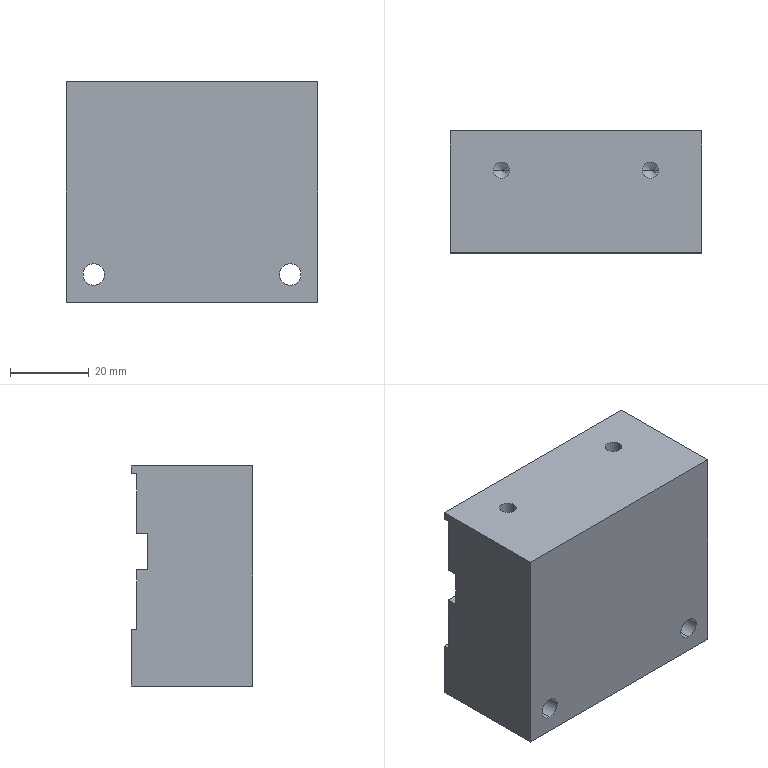Component | SolidWorks | JCT-03-01Base-1 | 1 solid | 32 faces | box 64 x 31 x 56 mm | volume 103150 mm3 | plane 16 | cylinder 12 | cone 4 | commonest cylinder face diameters 4.2 x4 10 x4 5.5 x4
build123d program:
from build123d import *

# Parameters (mm, degrees)
EXTRUDE1_DEPTH                                  = 32
M5_HEX_SOCKET_HEAD_CAP_SCREW_CBORE1_D           = 5.5
M5_HEX_SOCKET_HEAD_CAP_SCREW_CBORE1_CBORE_D     = 10
M5_HEX_SOCKET_HEAD_CAP_SCREW_CBORE1_CBORE_DEPTH = 6
M5_TAPPED_HOLE1_D                               = 4.2
M5_TAPPED_HOLE1_DEPTH                           = 12.4
M5_TAPPED_HOLE1_TIP                             = 1.262


with BuildPart() as part:
    # Sketch1 → Extrude1 (new, symmetric)
    with BuildSketch(Plane(origin=(0, 0, 0), x_dir=(0, 0, -1), z_dir=(1, 0, 0))):
        Polygon((0, 0), (-56, 0), (-56, 31), (-54, 31), (-54, 29.5), (-38.85, 29.5), (-38.85, 26.7), (-29.55, 26.7), (-29.55, 29.5), (-14.4, 29.5), (-14.4, 31), (0, 31), align=None)
    extrude(amount=EXTRUDE1_DEPTH, both=True)

    # M5 Hex Socket Head Cap Screw CBORE1 (through all)
    with Locations(Plane(origin=(0, 31, 0), x_dir=(-1, 0, 0), z_dir=(0, 1, 0))):
        with Locations((25, 7), (-25, 7)):
            CounterBoreHole(M5_HEX_SOCKET_HEAD_CAP_SCREW_CBORE1_D / 2, M5_HEX_SOCKET_HEAD_CAP_SCREW_CBORE1_CBORE_D / 2, M5_HEX_SOCKET_HEAD_CAP_SCREW_CBORE1_CBORE_DEPTH)

    # M5 Tapped Hole1
    with Locations(Plane.XY.offset(56)):
        with Locations((-19, 21), (19, 21)):
            Hole(M5_TAPPED_HOLE1_D / 2, depth=M5_TAPPED_HOLE1_DEPTH)
            with Locations((0, 0, -(M5_TAPPED_HOLE1_DEPTH + M5_TAPPED_HOLE1_TIP / 2))):  # 118° drill point
                Cone(0, M5_TAPPED_HOLE1_D / 2, M5_TAPPED_HOLE1_TIP, mode=Mode.SUBTRACT)


solid = part.part

# Placed as in the assembly
solid = solid.moved(Location((4.266, -17.701, 0), (0, 0, 0)))
STEP:
#1=COLOUR_RGB('',0.7922,0.8196,0.9333);
#2=FILL_AREA_STYLE_COLOUR('',#1);
#3=FILL_AREA_STYLE('',(#2));
#4=SURFACE_STYLE_FILL_AREA(#3);
#5=SURFACE_SIDE_STYLE('',(#4));
#6=SURFACE_STYLE_USAGE(.BOTH.,#5);
#7=PRESENTATION_STYLE_ASSIGNMENT((#6));
#8=CARTESIAN_POINT('',(-0.6627,0.1299,1.717));
#9=VERTEX_POINT('',#8);
#10=CARTESIAN_POINT('',(-0.4974,0.1299,1.717));
#11=VERTEX_POINT('',#10);
#12=CARTESIAN_POINT('',(-0.5801,0.1299,1.717));
#13=DIRECTION('',(0.,0.,1.));
#14=DIRECTION('',(1.,0.,0.));
#15=AXIS2_PLACEMENT_3D('',#12,#13,#14);
#16=CIRCLE('',#15,0.08268);
#17=EDGE_CURVE('',#9,#11,#16,.T.);
#18=ORIENTED_EDGE('',*,*,#17,.F.);
#19=CARTESIAN_POINT('',(-0.6627,0.1299,2.205));
#20=VERTEX_POINT('',#19);
#21=CARTESIAN_POINT('',(-0.6627,0.1299,2.205));
#22=DIRECTION('',(0.,0.,1.));
#23=VECTOR('',#22,39.37);
#24=LINE('',#21,#23);
#25=EDGE_CURVE('',#9,#20,#24,.T.);
#26=ORIENTED_EDGE('',*,*,#25,.T.);
#27=CARTESIAN_POINT('',(-0.4974,0.1299,2.205));
#28=VERTEX_POINT('',#27);
#29=CARTESIAN_POINT('',(-0.5801,0.1299,2.205));
#30=DIRECTION('',(0.,0.,1.));
#31=DIRECTION('',(1.,0.,0.));
#32=AXIS2_PLACEMENT_3D('',#29,#30,#31);
#33=CIRCLE('',#32,0.08268);
#34=EDGE_CURVE('',#20,#28,#33,.T.);
#35=ORIENTED_EDGE('',*,*,#34,.T.);
#36=CARTESIAN_POINT('',(-0.4974,0.1299,2.205));
#37=DIRECTION('',(0.,0.,1.));
#38=VECTOR('',#37,39.37);
#39=LINE('',#36,#38);
#40=EDGE_CURVE('',#11,#28,#39,.T.);
#41=ORIENTED_EDGE('',*,*,#40,.F.);
#42=EDGE_LOOP('',(#18,#26,#35,#41));
#43=FACE_OUTER_BOUND('',#42,.T.);
#44=CARTESIAN_POINT('',(-0.5801,0.1299,2.205));
#45=DIRECTION('',(0.,0.,1.));
#46=DIRECTION('',(1.,0.,0.));
#47=AXIS2_PLACEMENT_3D('',#44,#45,#46);
#48=CYLINDRICAL_SURFACE('',#47,0.08268);
#49=ADVANCED_FACE('',(#43),#48,.F.);
#50=CARTESIAN_POINT('',(-0.5801,0.1299,1.667));
#51=VERTEX_POINT('',#50);
#52=CARTESIAN_POINT('',(-0.4974,0.1299,1.717));
#53=DIRECTION('',(0.8572,0.,0.515));
#54=VECTOR('',#53,39.37);
#55=LINE('',#52,#54);
#56=EDGE_CURVE('',#51,#11,#55,.T.);
#57=ORIENTED_EDGE('',*,*,#56,.F.);
#58=CARTESIAN_POINT('',(-0.6627,0.1299,1.717));
#59=DIRECTION('',(-0.8572,0.,0.515));
#60=VECTOR('',#59,39.37);
#61=LINE('',#58,#60);
#62=EDGE_CURVE('',#51,#9,#61,.T.);
#63=ORIENTED_EDGE('',*,*,#62,.T.);
#64=ORIENTED_EDGE('',*,*,#17,.T.);
#65=EDGE_LOOP('',(#57,#63,#64));
#66=FACE_OUTER_BOUND('',#65,.T.);
#67=CARTESIAN_POINT('',(-0.5801,0.1299,1.717));
#68=DIRECTION('',(0.,0.,1.));
#69=DIRECTION('',(1.,0.,0.));
#70=AXIS2_PLACEMENT_3D('',#67,#68,#69);
#71=CONICAL_SURFACE('',#70,0.08268,1.03);
#72=ADVANCED_FACE('',(#66),#71,.F.);
#73=CARTESIAN_POINT('',(0.8333,0.1299,1.717));
#74=VERTEX_POINT('',#73);
#75=CARTESIAN_POINT('',(0.9987,0.1299,1.717));
#76=VERTEX_POINT('',#75);
#77=CARTESIAN_POINT('',(0.916,0.1299,1.717));
#78=DIRECTION('',(0.,0.,1.));
#79=DIRECTION('',(1.,0.,0.));
#80=AXIS2_PLACEMENT_3D('',#77,#78,#79);
#81=CIRCLE('',#80,0.08268);
#82=EDGE_CURVE('',#74,#76,#81,.T.);
#83=ORIENTED_EDGE('',*,*,#82,.F.);
#84=CARTESIAN_POINT('',(0.8333,0.1299,2.205));
#85=VERTEX_POINT('',#84);
#86=CARTESIAN_POINT('',(0.8333,0.1299,2.205));
#87=DIRECTION('',(0.,0.,1.));
#88=VECTOR('',#87,39.37);
#89=LINE('',#86,#88);
#90=EDGE_CURVE('',#74,#85,#89,.T.);
#91=ORIENTED_EDGE('',*,*,#90,.T.);
#92=CARTESIAN_POINT('',(0.9987,0.1299,2.205));
#93=VERTEX_POINT('',#92);
#94=CARTESIAN_POINT('',(0.916,0.1299,2.205));
#95=DIRECTION('',(0.,0.,1.));
#96=DIRECTION('',(1.,0.,0.));
#97=AXIS2_PLACEMENT_3D('',#94,#95,#96);
#98=CIRCLE('',#97,0.08268);
#99=EDGE_CURVE('',#85,#93,#98,.T.);
#100=ORIENTED_EDGE('',*,*,#99,.T.);
#101=CARTESIAN_POINT('',(0.9987,0.1299,2.205));
#102=DIRECTION('',(0.,0.,1.));
#103=VECTOR('',#102,39.37);
#104=LINE('',#101,#103);
#105=EDGE_CURVE('',#76,#93,#104,.T.);
#106=ORIENTED_EDGE('',*,*,#105,.F.);
#107=EDGE_LOOP('',(#83,#91,#100,#106));
#108=FACE_OUTER_BOUND('',#107,.T.);
#109=CARTESIAN_POINT('',(0.916,0.1299,2.205));
#110=DIRECTION('',(0.,0.,1.));
#111=DIRECTION('',(1.,0.,0.));
#112=AXIS2_PLACEMENT_3D('',#109,#110,#111);
#113=CYLINDRICAL_SURFACE('',#112,0.08268);
#114=ADVANCED_FACE('',(#108),#113,.F.);
#115=CARTESIAN_POINT('',(0.916,0.1299,1.667));
#116=VERTEX_POINT('',#115);
#117=CARTESIAN_POINT('',(0.9987,0.1299,1.717));
#118=DIRECTION('',(0.8572,0.,0.515));
#119=VECTOR('',#118,39.37);
#120=LINE('',#117,#119);
#121=EDGE_CURVE('',#116,#76,#120,.T.);
#122=ORIENTED_EDGE('',*,*,#121,.F.);
#123=CARTESIAN_POINT('',(0.8333,0.1299,1.717));
#124=DIRECTION('',(-0.8572,0.,0.515));
#125=VECTOR('',#124,39.37);
#126=LINE('',#123,#125);
#127=EDGE_CURVE('',#116,#74,#126,.T.);
#128=ORIENTED_EDGE('',*,*,#127,.T.);
#129=ORIENTED_EDGE('',*,*,#82,.T.);
#130=EDGE_LOOP('',(#122,#128,#129));
#131=FACE_OUTER_BOUND('',#130,.T.);
#132=CARTESIAN_POINT('',(0.916,0.1299,1.717));
#133=DIRECTION('',(0.,0.,1.));
#134=DIRECTION('',(1.,0.,0.));
#135=AXIS2_PLACEMENT_3D('',#132,#133,#134);
#136=CONICAL_SURFACE('',#135,0.08268,1.03);
#137=ADVANCED_FACE('',(#131),#136,.F.);
#138=CARTESIAN_POINT('',(-0.8163,0.2874,0.07874));
#139=VERTEX_POINT('',#138);
#140=CARTESIAN_POINT('',(-0.8163,0.2874,0.4724));
#141=VERTEX_POINT('',#140);
#142=CARTESIAN_POINT('',(-0.8163,0.2874,0.2756));
#143=DIRECTION('',(0.,1.,-0.));
#144=DIRECTION('',(0.,0.,1.));
#145=AXIS2_PLACEMENT_3D('',#142,#143,#144);
#146=CIRCLE('',#145,0.1969);
#147=EDGE_CURVE('',#139,#141,#146,.T.);
#148=ORIENTED_EDGE('',*,*,#147,.F.);
#149=CARTESIAN_POINT('',(-0.8163,0.5236,0.07874));
#150=VERTEX_POINT('',#149);
#151=CARTESIAN_POINT('',(-0.8163,0.5236,0.07874));
#152=DIRECTION('',(0.,1.,-0.));
#153=VECTOR('',#152,39.37);
#154=LINE('',#151,#153);
#155=EDGE_CURVE('',#139,#150,#154,.T.);
#156=ORIENTED_EDGE('',*,*,#155,.T.);
#157=CARTESIAN_POINT('',(-0.8163,0.5236,0.4724));
#158=VERTEX_POINT('',#157);
#159=CARTESIAN_POINT('',(-0.8163,0.5236,0.2756));
#160=DIRECTION('',(0.,1.,-0.));
#161=DIRECTION('',(0.,0.,1.));
#162=AXIS2_PLACEMENT_3D('',#159,#160,#161);
#163=CIRCLE('',#162,0.1969);
#164=EDGE_CURVE('',#150,#158,#163,.T.);
#165=ORIENTED_EDGE('',*,*,#164,.T.);
#166=CARTESIAN_POINT('',(-0.8163,0.5236,0.4724));
#167=DIRECTION('',(0.,1.,-0.));
#168=VECTOR('',#167,39.37);
#169=LINE('',#166,#168);
#170=EDGE_CURVE('',#141,#158,#169,.T.);
#171=ORIENTED_EDGE('',*,*,#170,.F.);
#172=EDGE_LOOP('',(#148,#156,#165,#171));
#173=FACE_OUTER_BOUND('',#172,.T.);
#174=CARTESIAN_POINT('',(-0.8163,0.5236,0.2756));
#175=DIRECTION('',(0.,1.,-0.));
#176=DIRECTION('',(0.,0.,1.));
#177=AXIS2_PLACEMENT_3D('',#174,#175,#176);
#178=CYLINDRICAL_SURFACE('',#177,0.1969);
#179=ADVANCED_FACE('',(#173),#178,.F.);
#180=CARTESIAN_POINT('',(-0.8163,-0.6969,0.1673));
#181=VERTEX_POINT('',#180);
#182=CARTESIAN_POINT('',(-0.8163,-0.6969,0.3839));
#183=VERTEX_POINT('',#182);
#184=CARTESIAN_POINT('',(-0.8163,-0.6969,0.2756));
#185=DIRECTION('',(0.,1.,-0.));
#186=DIRECTION('',(0.,0.,1.));
#187=AXIS2_PLACEMENT_3D('',#184,#185,#186);
#188=CIRCLE('',#187,0.1083);
#189=EDGE_CURVE('',#181,#183,#188,.T.);
#190=ORIENTED_EDGE('',*,*,#189,.F.);
#191=CARTESIAN_POINT('',(-0.8163,0.2874,0.1673));
#192=VERTEX_POINT('',#191);
#193=CARTESIAN_POINT('',(-0.8163,0.5236,0.1673));
#194=DIRECTION('',(0.,1.,-0.));
#195=VECTOR('',#194,39.37);
#196=LINE('',#193,#195);
#197=EDGE_CURVE('',#181,#192,#196,.T.);
#198=ORIENTED_EDGE('',*,*,#197,.T.);
#199=CARTESIAN_POINT('',(-0.8163,0.2874,0.3839));
#200=VERTEX_POINT('',#199);
#201=CARTESIAN_POINT('',(-0.8163,0.2874,0.2756));
#202=DIRECTION('',(0.,1.,-0.));
#203=DIRECTION('',(0.,0.,1.));
#204=AXIS2_PLACEMENT_3D('',#201,#202,#203);
#205=CIRCLE('',#204,0.1083);
#206=EDGE_CURVE('',#192,#200,#205,.T.);
#207=ORIENTED_EDGE('',*,*,#206,.T.);
#208=CARTESIAN_POINT('',(-0.8163,0.5236,0.3839));
#209=DIRECTION('',(0.,1.,-0.));
#210=VECTOR('',#209,39.37);
#211=LINE('',#208,#210);
#212=EDGE_CURVE('',#183,#200,#211,.T.);
#213=ORIENTED_EDGE('',*,*,#212,.F.);
#214=EDGE_LOOP('',(#190,#198,#207,#213));
#215=FACE_OUTER_BOUND('',#214,.T.);
#216=CARTESIAN_POINT('',(-0.8163,0.5236,0.2756));
#217=DIRECTION('',(0.,1.,-0.));
#218=DIRECTION('',(0.,0.,1.));
#219=AXIS2_PLACEMENT_3D('',#216,#217,#218);
#220=CYLINDRICAL_SURFACE('',#219,0.1083);
#221=ADVANCED_FACE('',(#215),#220,.F.);
#222=CARTESIAN_POINT('',(1.152,0.2874,0.07874));
#223=VERTEX_POINT('',#222);
#224=CARTESIAN_POINT('',(1.152,0.2874,0.4724));
#225=VERTEX_POINT('',#224);
#226=CARTESIAN_POINT('',(1.152,0.2874,0.2756));
#227=DIRECTION('',(0.,1.,-0.));
#228=DIRECTION('',(0.,0.,1.));
#229=AXIS2_PLACEMENT_3D('',#226,#227,#228);
#230=CIRCLE('',#229,0.1969);
#231=EDGE_CURVE('',#223,#225,#230,.T.);
#232=ORIENTED_EDGE('',*,*,#231,.F.);
#233=CARTESIAN_POINT('',(1.152,0.5236,0.07874));
#234=VERTEX_POINT('',#233);
#235=CARTESIAN_POINT('',(1.152,0.5236,0.07874));
#236=DIRECTION('',(0.,1.,-0.));
#237=VECTOR('',#236,39.37);
#238=LINE('',#235,#237);
#239=EDGE_CURVE('',#223,#234,#238,.T.);
#240=ORIENTED_EDGE('',*,*,#239,.T.);
#241=CARTESIAN_POINT('',(1.152,0.5236,0.4724));
#242=VERTEX_POINT('',#241);
#243=CARTESIAN_POINT('',(1.152,0.5236,0.2756));
#244=DIRECTION('',(0.,1.,-0.));
#245=DIRECTION('',(0.,0.,1.));
#246=AXIS2_PLACEMENT_3D('',#243,#244,#245);
#247=CIRCLE('',#246,0.1969);
#248=EDGE_CURVE('',#234,#242,#247,.T.);
#249=ORIENTED_EDGE('',*,*,#248,.T.);
#250=CARTESIAN_POINT('',(1.152,0.5236,0.4724));
#251=DIRECTION('',(0.,1.,-0.));
#252=VECTOR('',#251,39.37);
#253=LINE('',#250,#252);
#254=EDGE_CURVE('',#225,#242,#253,.T.);
#255=ORIENTED_EDGE('',*,*,#254,.F.);
#256=EDGE_LOOP('',(#232,#240,#249,#255));
#257=FACE_OUTER_BOUND('',#256,.T.);
#258=CARTESIAN_POINT('',(1.152,0.5236,0.2756));
#259=DIRECTION('',(0.,1.,-0.));
#260=DIRECTION('',(0.,0.,1.));
#261=AXIS2_PLACEMENT_3D('',#258,#259,#260);
#262=CYLINDRICAL_SURFACE('',#261,0.1969);
#263=ADVANCED_FACE('',(#257),#262,.F.);
#264=CARTESIAN_POINT('',(1.152,-0.6969,0.1673));
#265=VERTEX_POINT('',#264);
#266=CARTESIAN_POINT('',(1.152,-0.6969,0.3839));
#267=VERTEX_POINT('',#266);
#268=CARTESIAN_POINT('',(1.152,-0.6969,0.2756));
#269=DIRECTION('',(0.,1.,-0.));
#270=DIRECTION('',(0.,0.,1.));
#271=AXIS2_PLACEMENT_3D('',#268,#269,#270);
#272=CIRCLE('',#271,0.1083);
#273=EDGE_CURVE('',#265,#267,#272,.T.);
#274=ORIENTED_EDGE('',*,*,#273,.F.);
#275=CARTESIAN_POINT('',(1.152,0.2874,0.1673));
#276=VERTEX_POINT('',#275);
#277=CARTESIAN_POINT('',(1.152,0.5236,0.1673));
#278=DIRECTION('',(0.,1.,-0.));
#279=VECTOR('',#278,39.37);
#280=LINE('',#277,#279);
#281=EDGE_CURVE('',#265,#276,#280,.T.);
#282=ORIENTED_EDGE('',*,*,#281,.T.);
#283=CARTESIAN_POINT('',(1.152,0.2874,0.3839));
#284=VERTEX_POINT('',#283);
#285=CARTESIAN_POINT('',(1.152,0.2874,0.2756));
#286=DIRECTION('',(0.,1.,-0.));
#287=DIRECTION('',(0.,0.,1.));
#288=AXIS2_PLACEMENT_3D('',#285,#286,#287);
#289=CIRCLE('',#288,0.1083);
#290=EDGE_CURVE('',#276,#284,#289,.T.);
#291=ORIENTED_EDGE('',*,*,#290,.T.);
#292=CARTESIAN_POINT('',(1.152,0.5236,0.3839));
#293=DIRECTION('',(0.,1.,-0.));
#294=VECTOR('',#293,39.37);
#295=LINE('',#292,#294);
#296=EDGE_CURVE('',#267,#284,#295,.T.);
#297=ORIENTED_EDGE('',*,*,#296,.F.);
#298=EDGE_LOOP('',(#274,#282,#291,#297));
#299=FACE_OUTER_BOUND('',#298,.T.);
#300=CARTESIAN_POINT('',(1.152,0.5236,0.2756));
#301=DIRECTION('',(0.,1.,-0.));
#302=DIRECTION('',(0.,0.,1.));
#303=AXIS2_PLACEMENT_3D('',#300,#301,#302);
#304=CYLINDRICAL_SURFACE('',#303,0.1083);
#305=ADVANCED_FACE('',(#299),#304,.F.);
#306=CARTESIAN_POINT('',(-1.092,-0.6969,0.));
#307=VERTEX_POINT('',#306);
#308=CARTESIAN_POINT('',(-1.092,0.5236,0.));
#309=VERTEX_POINT('',#308);
#310=CARTESIAN_POINT('',(-1.092,0.5236,0.));
#311=DIRECTION('',(0.,1.,0.));
#312=VECTOR('',#311,39.37);
#313=LINE('',#310,#312);
#314=EDGE_CURVE('',#307,#309,#313,.T.);
#315=ORIENTED_EDGE('',*,*,#314,.T.);
#316=CARTESIAN_POINT('',(1.428,0.5236,0.));
#317=VERTEX_POINT('',#316);
#318=CARTESIAN_POINT('',(1.428,0.5236,0.));
#319=DIRECTION('',(-1.,0.,0.));
#320=VECTOR('',#319,39.37);
#321=LINE('',#318,#320);
#322=EDGE_CURVE('',#317,#309,#321,.T.);
#323=ORIENTED_EDGE('',*,*,#322,.F.);
#324=CARTESIAN_POINT('',(1.428,-0.6969,0.));
#325=VERTEX_POINT('',#324);
#326=CARTESIAN_POINT('',(1.428,0.5236,0.));
#327=DIRECTION('',(0.,1.,0.));
#328=VECTOR('',#327,39.37);
#329=LINE('',#326,#328);
#330=EDGE_CURVE('',#325,#317,#329,.T.);
#331=ORIENTED_EDGE('',*,*,#330,.F.);
#332=CARTESIAN_POINT('',(1.428,-0.6969,0.));
#333=DIRECTION('',(-1.,0.,0.));
#334=VECTOR('',#333,39.37);
#335=LINE('',#332,#334);
#336=EDGE_CURVE('',#325,#307,#335,.T.);
#337=ORIENTED_EDGE('',*,*,#336,.T.);
#338=EDGE_LOOP('',(#315,#323,#331,#337));
#339=FACE_OUTER_BOUND('',#338,.T.);
#340=CARTESIAN_POINT('',(1.428,0.5236,0.));
#341=DIRECTION('',(0.,-0.,1.));
#342=DIRECTION('',(0.,-1.,-0.));
#343=AXIS2_PLACEMENT_3D('',#340,#341,#342);
#344=PLANE('',#343);
#345=ADVANCED_FACE('',(#339),#344,.F.);
#346=CARTESIAN_POINT('',(-0.8163,0.5236,0.2756));
#347=DIRECTION('',(0.,1.,-0.));
#348=DIRECTION('',(0.,0.,1.));
#349=AXIS2_PLACEMENT_3D('',#346,#347,#348);
#350=CIRCLE('',#349,0.1969);
#351=EDGE_CURVE('',#158,#150,#350,.T.);
#352=ORIENTED_EDGE('',*,*,#351,.F.);
#353=ORIENTED_EDGE('',*,*,#164,.F.);
#354=EDGE_LOOP('',(#352,#353));
#355=FACE_BOUND('',#354,.T.);
#356=CARTESIAN_POINT('',(1.152,0.5236,0.2756));
#357=DIRECTION('',(0.,1.,-0.));
#358=DIRECTION('',(0.,0.,1.));
#359=AXIS2_PLACEMENT_3D('',#356,#357,#358);
#360=CIRCLE('',#359,0.1969);
#361=EDGE_CURVE('',#242,#234,#360,.T.);
#362=ORIENTED_EDGE('',*,*,#361,.F.);
#363=ORIENTED_EDGE('',*,*,#248,.F.);
#364=EDGE_LOOP('',(#362,#363));
#365=FACE_BOUND('',#364,.T.);
#366=CARTESIAN_POINT('',(-1.092,0.5236,0.5669));
#367=VERTEX_POINT('',#366);
#368=CARTESIAN_POINT('',(-1.092,0.5236,0.5669));
#369=DIRECTION('',(0.,0.,1.));
#370=VECTOR('',#369,39.37);
#371=LINE('',#368,#370);
#372=EDGE_CURVE('',#309,#367,#371,.T.);
#373=ORIENTED_EDGE('',*,*,#372,.T.);
#374=CARTESIAN_POINT('',(1.428,0.5236,0.5669));
#375=VERTEX_POINT('',#374);
#376=CARTESIAN_POINT('',(1.428,0.5236,0.5669));
#377=DIRECTION('',(-1.,0.,0.));
#378=VECTOR('',#377,39.37);
#379=LINE('',#376,#378);
#380=EDGE_CURVE('',#375,#367,#379,.T.);
#381=ORIENTED_EDGE('',*,*,#380,.F.);
#382=CARTESIAN_POINT('',(1.428,0.5236,0.5669));
#383=DIRECTION('',(0.,0.,1.));
#384=VECTOR('',#383,39.37);
#385=LINE('',#382,#384);
#386=EDGE_CURVE('',#317,#375,#385,.T.);
#387=ORIENTED_EDGE('',*,*,#386,.F.);
#388=ORIENTED_EDGE('',*,*,#322,.T.);
#389=EDGE_LOOP('',(#373,#381,#387,#388));
#390=FACE_OUTER_BOUND('',#389,.T.);
#391=CARTESIAN_POINT('',(1.428,0.5236,0.5669));
#392=DIRECTION('',(0.,-1.,0.));
#393=DIRECTION('',(0.,-0.,-1.));
#394=AXIS2_PLACEMENT_3D('',#391,#392,#393);
#395=PLANE('',#394);
#396=ADVANCED_FACE('',(#355,#365,#390),#395,.F.);
#397=CARTESIAN_POINT('',(-1.092,0.4645,0.5669));
#398=VERTEX_POINT('',#397);
#399=CARTESIAN_POINT('',(-1.092,0.4645,0.5669));
#400=DIRECTION('',(0.,-1.,0.));
#401=VECTOR('',#400,39.37);
#402=LINE('',#399,#401);
#403=EDGE_CURVE('',#367,#398,#402,.T.);
#404=ORIENTED_EDGE('',*,*,#403,.T.);
#405=CARTESIAN_POINT('',(1.428,0.4645,0.5669));
#406=VERTEX_POINT('',#405);
#407=CARTESIAN_POINT('',(1.428,0.4645,0.5669));
#408=DIRECTION('',(-1.,0.,0.));
#409=VECTOR('',#408,39.37);
#410=LINE('',#407,#409);
#411=EDGE_CURVE('',#406,#398,#410,.T.);
#412=ORIENTED_EDGE('',*,*,#411,.F.);
#413=CARTESIAN_POINT('',(1.428,0.4645,0.5669));
#414=DIRECTION('',(0.,-1.,0.));
#415=VECTOR('',#414,39.37);
#416=LINE('',#413,#415);
#417=EDGE_CURVE('',#375,#406,#416,.T.);
#418=ORIENTED_EDGE('',*,*,#417,.F.);
#419=ORIENTED_EDGE('',*,*,#380,.T.);
#420=EDGE_LOOP('',(#404,#412,#418,#419));
#421=FACE_OUTER_BOUND('',#420,.T.);
#422=CARTESIAN_POINT('',(1.428,0.4645,0.5669));
#423=DIRECTION('',(0.,-0.,-1.));
#424=DIRECTION('',(0.,1.,-0.));
#425=AXIS2_PLACEMENT_3D('',#422,#423,#424);
#426=PLANE('',#425);
#427=ADVANCED_FACE('',(#421),#426,.F.);
#428=CARTESIAN_POINT('',(-1.092,0.4645,1.163));
#429=VERTEX_POINT('',#428);
#430=CARTESIAN_POINT('',(-1.092,0.4645,1.163));
#431=DIRECTION('',(0.,-0.,1.));
#432=VECTOR('',#431,39.37);
#433=LINE('',#430,#432);
#434=EDGE_CURVE('',#398,#429,#433,.T.);
#435=ORIENTED_EDGE('',*,*,#434,.T.);
#436=CARTESIAN_POINT('',(1.428,0.4645,1.163));
#437=VERTEX_POINT('',#436);
#438=CARTESIAN_POINT('',(1.428,0.4645,1.163));
#439=DIRECTION('',(-1.,0.,0.));
#440=VECTOR('',#439,39.37);
#441=LINE('',#438,#440);
#442=EDGE_CURVE('',#437,#429,#441,.T.);
#443=ORIENTED_EDGE('',*,*,#442,.F.);
#444=CARTESIAN_POINT('',(1.428,0.4645,1.163));
#445=DIRECTION('',(0.,-0.,1.));
#446=VECTOR('',#445,39.37);
#447=LINE('',#444,#446);
#448=EDGE_CURVE('',#406,#437,#447,.T.);
#449=ORIENTED_EDGE('',*,*,#448,.F.);
#450=ORIENTED_EDGE('',*,*,#411,.T.);
#451=EDGE_LOOP('',(#435,#443,#449,#450));
#452=FACE_OUTER_BOUND('',#451,.T.);
#453=CARTESIAN_POINT('',(1.428,0.4645,1.163));
#454=DIRECTION('',(0.,-1.,-0.));
#455=DIRECTION('',(0.,0.,-1.));
#456=AXIS2_PLACEMENT_3D('',#453,#454,#455);
#457=PLANE('',#456);
#458=ADVANCED_FACE('',(#452),#457,.F.);
#459=CARTESIAN_POINT('',(-1.092,0.3543,1.163));
#460=VERTEX_POINT('',#459);
#461=CARTESIAN_POINT('',(-1.092,0.3543,1.163));
#462=DIRECTION('',(0.,-1.,0.));
#463=VECTOR('',#462,39.37);
#464=LINE('',#461,#463);
#465=EDGE_CURVE('',#429,#460,#464,.T.);
#466=ORIENTED_EDGE('',*,*,#465,.T.);
#467=CARTESIAN_POINT('',(1.428,0.3543,1.163));
#468=VERTEX_POINT('',#467);
#469=CARTESIAN_POINT('',(1.428,0.3543,1.163));
#470=DIRECTION('',(-1.,0.,0.));
#471=VECTOR('',#470,39.37);
#472=LINE('',#469,#471);
#473=EDGE_CURVE('',#468,#460,#472,.T.);
#474=ORIENTED_EDGE('',*,*,#473,.F.);
#475=CARTESIAN_POINT('',(1.428,0.3543,1.163));
#476=DIRECTION('',(0.,-1.,0.));
#477=VECTOR('',#476,39.37);
#478=LINE('',#475,#477);
#479=EDGE_CURVE('',#437,#468,#478,.T.);
#480=ORIENTED_EDGE('',*,*,#479,.F.);
#481=ORIENTED_EDGE('',*,*,#442,.T.);
#482=EDGE_LOOP('',(#466,#474,#480,#481));
#483=FACE_OUTER_BOUND('',#482,.T.);
#484=CARTESIAN_POINT('',(1.428,0.3543,1.163));
#485=DIRECTION('',(0.,0.,-1.));
#486=DIRECTION('',(-1.,0.,0.));
#487=AXIS2_PLACEMENT_3D('',#484,#485,#486);
#488=PLANE('',#487);
#489=ADVANCED_FACE('',(#483),#488,.F.);
#490=CARTESIAN_POINT('',(-1.092,0.3543,1.53));
#491=VERTEX_POINT('',#490);
#492=CARTESIAN_POINT('',(-1.092,0.3543,1.53));
#493=DIRECTION('',(0.,0.,1.));
#494=VECTOR('',#493,39.37);
#495=LINE('',#492,#494);
#496=EDGE_CURVE('',#460,#491,#495,.T.);
#497=ORIENTED_EDGE('',*,*,#496,.T.);
#498=CARTESIAN_POINT('',(1.428,0.3543,1.53));
#499=VERTEX_POINT('',#498);
#500=CARTESIAN_POINT('',(1.428,0.3543,1.53));
#501=DIRECTION('',(-1.,0.,0.));
#502=VECTOR('',#501,39.37);
#503=LINE('',#500,#502);
#504=EDGE_CURVE('',#499,#491,#503,.T.);
#505=ORIENTED_EDGE('',*,*,#504,.F.);
#506=CARTESIAN_POINT('',(1.428,0.3543,1.53));
#507=DIRECTION('',(0.,0.,1.));
#508=VECTOR('',#507,39.37);
#509=LINE('',#506,#508);
#510=EDGE_CURVE('',#468,#499,#509,.T.);
#511=ORIENTED_EDGE('',*,*,#510,.F.);
#512=ORIENTED_EDGE('',*,*,#473,.T.);
#513=EDGE_LOOP('',(#497,#505,#511,#512));
#514=FACE_OUTER_BOUND('',#513,.T.);
#515=CARTESIAN_POINT('',(1.428,0.3543,1.53));
#516=DIRECTION('',(0.,-1.,0.));
#517=DIRECTION('',(0.,0.,-1.));
#518=AXIS2_PLACEMENT_3D('',#515,#516,#517);
#519=PLANE('',#518);
#520=ADVANCED_FACE('',(#514),#519,.F.);
#521=CARTESIAN_POINT('',(-1.092,0.4645,1.53));
#522=VERTEX_POINT('',#521);
#523=CARTESIAN_POINT('',(-1.092,0.4645,1.53));
#524=DIRECTION('',(0.,1.,0.));
#525=VECTOR('',#524,39.37);
#526=LINE('',#523,#525);
#527=EDGE_CURVE('',#491,#522,#526,.T.);
#528=ORIENTED_EDGE('',*,*,#527,.T.);
#529=CARTESIAN_POINT('',(1.428,0.4645,1.53));
#530=VERTEX_POINT('',#529);
#531=CARTESIAN_POINT('',(1.428,0.4645,1.53));
#532=DIRECTION('',(-1.,0.,0.));
#533=VECTOR('',#532,39.37);
#534=LINE('',#531,#533);
#535=EDGE_CURVE('',#530,#522,#534,.T.);
#536=ORIENTED_EDGE('',*,*,#535,.F.);
#537=CARTESIAN_POINT('',(1.428,0.4645,1.53));
#538=DIRECTION('',(0.,1.,0.));
#539=VECTOR('',#538,39.37);
#540=LINE('',#537,#539);
#541=EDGE_CURVE('',#499,#530,#540,.T.);
#542=ORIENTED_EDGE('',*,*,#541,.F.);
#543=ORIENTED_EDGE('',*,*,#504,.T.);
#544=EDGE_LOOP('',(#528,#536,#542,#543));
#545=FACE_OUTER_BOUND('',#544,.T.);
#546=CARTESIAN_POINT('',(1.428,0.4645,1.53));
#547=DIRECTION('',(0.,0.,1.));
#548=DIRECTION('',(1.,0.,0.));
#549=AXIS2_PLACEMENT_3D('',#546,#547,#548);
#550=PLANE('',#549);
#551=ADVANCED_FACE('',(#545),#550,.F.);
#552=CARTESIAN_POINT('',(-1.092,0.4645,2.126));
#553=VERTEX_POINT('',#552);
#554=CARTESIAN_POINT('',(-1.092,0.4645,2.126));
#555=DIRECTION('',(0.,0.,1.));
#556=VECTOR('',#555,39.37);
#557=LINE('',#554,#556);
#558=EDGE_CURVE('',#522,#553,#557,.T.);
#559=ORIENTED_EDGE('',*,*,#558,.T.);
#560=CARTESIAN_POINT('',(1.428,0.4645,2.126));
#561=VERTEX_POINT('',#560);
#562=CARTESIAN_POINT('',(1.428,0.4645,2.126));
#563=DIRECTION('',(-1.,0.,0.));
#564=VECTOR('',#563,39.37);
#565=LINE('',#562,#564);
#566=EDGE_CURVE('',#561,#553,#565,.T.);
#567=ORIENTED_EDGE('',*,*,#566,.F.);
#568=CARTESIAN_POINT('',(1.428,0.4645,2.126));
#569=DIRECTION('',(0.,0.,1.));
#570=VECTOR('',#569,39.37);
#571=LINE('',#568,#570);
#572=EDGE_CURVE('',#530,#561,#571,.T.);
#573=ORIENTED_EDGE('',*,*,#572,.F.);
#574=ORIENTED_EDGE('',*,*,#535,.T.);
#575=EDGE_LOOP('',(#559,#567,#573,#574));
#576=FACE_OUTER_BOUND('',#575,.T.);
#577=CARTESIAN_POINT('',(1.428,0.4645,2.126));
#578=DIRECTION('',(0.,-1.,0.));
#579=DIRECTION('',(0.,0.,-1.));
#580=AXIS2_PLACEMENT_3D('',#577,#578,#579);
#581=PLANE('',#580);
#582=ADVANCED_FACE('',(#576),#581,.F.);
#583=CARTESIAN_POINT('',(-1.092,0.5236,2.126));
#584=VERTEX_POINT('',#583);
#585=CARTESIAN_POINT('',(-1.092,0.5236,2.126));
#586=DIRECTION('',(0.,1.,-0.));
#587=VECTOR('',#586,39.37);
#588=LINE('',#585,#587);
#589=EDGE_CURVE('',#553,#584,#588,.T.);
#590=ORIENTED_EDGE('',*,*,#589,.T.);
#591=CARTESIAN_POINT('',(1.428,0.5236,2.126));
#592=VERTEX_POINT('',#591);
#593=CARTESIAN_POINT('',(1.428,0.5236,2.126));
#594=DIRECTION('',(-1.,0.,0.));
#595=VECTOR('',#594,39.37);
#596=LINE('',#593,#595);
#597=EDGE_CURVE('',#592,#584,#596,.T.);
#598=ORIENTED_EDGE('',*,*,#597,.F.);
#599=CARTESIAN_POINT('',(1.428,0.5236,2.126));
#600=DIRECTION('',(0.,1.,-0.));
#601=VECTOR('',#600,39.37);
#602=LINE('',#599,#601);
#603=EDGE_CURVE('',#561,#592,#602,.T.);
#604=ORIENTED_EDGE('',*,*,#603,.F.);
#605=ORIENTED_EDGE('',*,*,#566,.T.);
#606=EDGE_LOOP('',(#590,#598,#604,#605));
#607=FACE_OUTER_BOUND('',#606,.T.);
#608=CARTESIAN_POINT('',(1.428,0.5236,2.126));
#609=DIRECTION('',(0.,0.,1.));
#610=DIRECTION('',(0.,-1.,0.));
#611=AXIS2_PLACEMENT_3D('',#608,#609,#610);
#612=PLANE('',#611);
#613=ADVANCED_FACE('',(#607),#612,.F.);
#614=CARTESIAN_POINT('',(-1.092,0.5236,2.205));
#615=VERTEX_POINT('',#614);
#616=CARTESIAN_POINT('',(-1.092,0.5236,2.205));
#617=DIRECTION('',(0.,-0.,1.));
#618=VECTOR('',#617,39.37);
#619=LINE('',#616,#618);
#620=EDGE_CURVE('',#584,#615,#619,.T.);
#621=ORIENTED_EDGE('',*,*,#620,.T.);
#622=CARTESIAN_POINT('',(1.428,0.5236,2.205));
#623=VERTEX_POINT('',#622);
#624=CARTESIAN_POINT('',(1.428,0.5236,2.205));
#625=DIRECTION('',(-1.,0.,0.));
#626=VECTOR('',#625,39.37);
#627=LINE('',#624,#626);
#628=EDGE_CURVE('',#623,#615,#627,.T.);
#629=ORIENTED_EDGE('',*,*,#628,.F.);
#630=CARTESIAN_POINT('',(1.428,0.5236,2.205));
#631=DIRECTION('',(0.,-0.,1.));
#632=VECTOR('',#631,39.37);
#633=LINE('',#630,#632);
#634=EDGE_CURVE('',#592,#623,#633,.T.);
#635=ORIENTED_EDGE('',*,*,#634,.F.);
#636=ORIENTED_EDGE('',*,*,#597,.T.);
#637=EDGE_LOOP('',(#621,#629,#635,#636));
#638=FACE_OUTER_BOUND('',#637,.T.);
#639=CARTESIAN_POINT('',(1.428,0.5236,2.205));
#640=DIRECTION('',(0.,-1.,-0.));
#641=DIRECTION('',(0.,0.,-1.));
#642=AXIS2_PLACEMENT_3D('',#639,#640,#641);
#643=PLANE('',#642);
#644=ADVANCED_FACE('',(#638),#643,.F.);
#645=CARTESIAN_POINT('',(-0.5801,0.1299,2.205));
#646=DIRECTION('',(0.,0.,1.));
#647=DIRECTION('',(1.,0.,0.));
#648=AXIS2_PLACEMENT_3D('',#645,#646,#647);
#649=CIRCLE('',#648,0.08268);
#650=EDGE_CURVE('',#28,#20,#649,.T.);
#651=ORIENTED_EDGE('',*,*,#650,.F.);
#652=ORIENTED_EDGE('',*,*,#34,.F.);
#653=EDGE_LOOP('',(#651,#652));
#654=FACE_BOUND('',#653,.T.);
#655=CARTESIAN_POINT('',(0.916,0.1299,2.205));
#656=DIRECTION('',(0.,0.,1.));
#657=DIRECTION('',(1.,0.,0.));
#658=AXIS2_PLACEMENT_3D('',#655,#656,#657);
#659=CIRCLE('',#658,0.08268);
#660=EDGE_CURVE('',#93,#85,#659,.T.);
#661=ORIENTED_EDGE('',*,*,#660,.F.);
#662=ORIENTED_EDGE('',*,*,#99,.F.);
#663=EDGE_LOOP('',(#661,#662));
#664=FACE_BOUND('',#663,.T.);
#665=CARTESIAN_POINT('',(-1.092,-0.6969,2.205));
#666=VERTEX_POINT('',#665);
#667=CARTESIAN_POINT('',(-1.092,-0.6969,2.205));
#668=DIRECTION('',(0.,-1.,0.));
#669=VECTOR('',#668,39.37);
#670=LINE('',#667,#669);
#671=EDGE_CURVE('',#615,#666,#670,.T.);
#672=ORIENTED_EDGE('',*,*,#671,.T.);
#673=CARTESIAN_POINT('',(1.428,-0.6969,2.205));
#674=VERTEX_POINT('',#673);
#675=CARTESIAN_POINT('',(1.428,-0.6969,2.205));
#676=DIRECTION('',(-1.,0.,0.));
#677=VECTOR('',#676,39.37);
#678=LINE('',#675,#677);
#679=EDGE_CURVE('',#674,#666,#678,.T.);
#680=ORIENTED_EDGE('',*,*,#679,.F.);
#681=CARTESIAN_POINT('',(1.428,-0.6969,2.205));
#682=DIRECTION('',(0.,-1.,0.));
#683=VECTOR('',#682,39.37);
#684=LINE('',#681,#683);
#685=EDGE_CURVE('',#623,#674,#684,.T.);
#686=ORIENTED_EDGE('',*,*,#685,.F.);
#687=ORIENTED_EDGE('',*,*,#628,.T.);
#688=EDGE_LOOP('',(#672,#680,#686,#687));
#689=FACE_OUTER_BOUND('',#688,.T.);
#690=CARTESIAN_POINT('',(1.428,-0.6969,2.205));
#691=DIRECTION('',(0.,0.,-1.));
#692=DIRECTION('',(-1.,0.,0.));
#693=AXIS2_PLACEMENT_3D('',#690,#691,#692);
#694=PLANE('',#693);
#695=ADVANCED_FACE('',(#654,#664,#689),#694,.F.);
#696=CARTESIAN_POINT('',(-0.8163,-0.6969,0.2756));
#697=DIRECTION('',(0.,1.,-0.));
#698=DIRECTION('',(0.,0.,1.));
#699=AXIS2_PLACEMENT_3D('',#696,#697,#698);
#700=CIRCLE('',#699,0.1083);
#701=EDGE_CURVE('',#183,#181,#700,.T.);
#702=ORIENTED_EDGE('',*,*,#701,.T.);
#703=ORIENTED_EDGE('',*,*,#189,.T.);
#704=EDGE_LOOP('',(#702,#703));
#705=FACE_BOUND('',#704,.T.);
#706=CARTESIAN_POINT('',(1.152,-0.6969,0.2756));
#707=DIRECTION('',(0.,1.,-0.));
#708=DIRECTION('',(0.,0.,1.));
#709=AXIS2_PLACEMENT_3D('',#706,#707,#708);
#710=CIRCLE('',#709,0.1083);
#711=EDGE_CURVE('',#267,#265,#710,.T.);
#712=ORIENTED_EDGE('',*,*,#711,.T.);
#713=ORIENTED_EDGE('',*,*,#273,.T.);
#714=EDGE_LOOP('',(#712,#713));
#715=FACE_BOUND('',#714,.T.);
#716=CARTESIAN_POINT('',(-1.092,-0.6969,0.));
#717=DIRECTION('',(0.,0.,-1.));
#718=VECTOR('',#717,39.37);
#719=LINE('',#716,#718);
#720=EDGE_CURVE('',#666,#307,#719,.T.);
#721=ORIENTED_EDGE('',*,*,#720,.T.);
#722=ORIENTED_EDGE('',*,*,#336,.F.);
#723=CARTESIAN_POINT('',(1.428,-0.6969,0.));
#724=DIRECTION('',(0.,0.,-1.));
#725=VECTOR('',#724,39.37);
#726=LINE('',#723,#725);
#727=EDGE_CURVE('',#674,#325,#726,.T.);
#728=ORIENTED_EDGE('',*,*,#727,.F.);
#729=ORIENTED_EDGE('',*,*,#679,.T.);
#730=EDGE_LOOP('',(#721,#722,#728,#729));
#731=FACE_OUTER_BOUND('',#730,.T.);
#732=CARTESIAN_POINT('',(1.428,-0.6969,0.));
#733=DIRECTION('',(0.,1.,0.));
#734=DIRECTION('',(0.,-0.,1.));
#735=AXIS2_PLACEMENT_3D('',#732,#733,#734);
#736=PLANE('',#735);
#737=ADVANCED_FACE('',(#705,#715,#731),#736,.F.);
#738=ORIENTED_EDGE('',*,*,#330,.T.);
#739=ORIENTED_EDGE('',*,*,#386,.T.);
#740=ORIENTED_EDGE('',*,*,#417,.T.);
#741=ORIENTED_EDGE('',*,*,#448,.T.);
#742=ORIENTED_EDGE('',*,*,#479,.T.);
#743=ORIENTED_EDGE('',*,*,#510,.T.);
#744=ORIENTED_EDGE('',*,*,#541,.T.);
#745=ORIENTED_EDGE('',*,*,#572,.T.);
#746=ORIENTED_EDGE('',*,*,#603,.T.);
#747=ORIENTED_EDGE('',*,*,#634,.T.);
#748=ORIENTED_EDGE('',*,*,#685,.T.);
#749=ORIENTED_EDGE('',*,*,#727,.T.);
#750=EDGE_LOOP('',(#738,#739,#740,#741,#742,#743,#744,#745,#746,#747,#748,#749));
#751=FACE_OUTER_BOUND('',#750,.T.);
#752=CARTESIAN_POINT('',(1.428,-0.6969,0.));
#753=DIRECTION('',(-1.,0.,0.));
#754=DIRECTION('',(0.,0.,1.));
#755=AXIS2_PLACEMENT_3D('',#752,#753,#754);
#756=PLANE('',#755);
#757=ADVANCED_FACE('',(#751),#756,.F.);
#758=ORIENTED_EDGE('',*,*,#314,.F.);
#759=ORIENTED_EDGE('',*,*,#720,.F.);
#760=ORIENTED_EDGE('',*,*,#671,.F.);
#761=ORIENTED_EDGE('',*,*,#620,.F.);
#762=ORIENTED_EDGE('',*,*,#589,.F.);
#763=ORIENTED_EDGE('',*,*,#558,.F.);
#764=ORIENTED_EDGE('',*,*,#527,.F.);
#765=ORIENTED_EDGE('',*,*,#496,.F.);
#766=ORIENTED_EDGE('',*,*,#465,.F.);
#767=ORIENTED_EDGE('',*,*,#434,.F.);
#768=ORIENTED_EDGE('',*,*,#403,.F.);
#769=ORIENTED_EDGE('',*,*,#372,.F.);
#770=EDGE_LOOP('',(#758,#759,#760,#761,#762,#763,#764,#765,#766,#767,#768,#769));
#771=FACE_OUTER_BOUND('',#770,.T.);
#772=CARTESIAN_POINT('',(-1.092,-0.6969,0.));
#773=DIRECTION('',(-1.,0.,0.));
#774=DIRECTION('',(0.,0.,1.));
#775=AXIS2_PLACEMENT_3D('',#772,#773,#774);
#776=PLANE('',#775);
#777=ADVANCED_FACE('',(#771),#776,.T.);
#778=ORIENTED_EDGE('',*,*,#281,.F.);
#779=ORIENTED_EDGE('',*,*,#711,.F.);
#780=ORIENTED_EDGE('',*,*,#296,.T.);
#781=CARTESIAN_POINT('',(1.152,0.2874,0.2756));
#782=DIRECTION('',(0.,1.,-0.));
#783=DIRECTION('',(0.,0.,1.));
#784=AXIS2_PLACEMENT_3D('',#781,#782,#783);
#785=CIRCLE('',#784,0.1083);
#786=EDGE_CURVE('',#284,#276,#785,.T.);
#787=ORIENTED_EDGE('',*,*,#786,.T.);
#788=EDGE_LOOP('',(#778,#779,#780,#787));
#789=FACE_OUTER_BOUND('',#788,.T.);
#790=CARTESIAN_POINT('',(1.152,0.5236,0.2756));
#791=DIRECTION('',(0.,1.,-0.));
#792=DIRECTION('',(0.,0.,1.));
#793=AXIS2_PLACEMENT_3D('',#790,#791,#792);
#794=CYLINDRICAL_SURFACE('',#793,0.1083);
#795=ADVANCED_FACE('',(#789),#794,.F.);
#796=ORIENTED_EDGE('',*,*,#786,.F.);
#797=ORIENTED_EDGE('',*,*,#290,.F.);
#798=EDGE_LOOP('',(#796,#797));
#799=FACE_BOUND('',#798,.T.);
#800=CARTESIAN_POINT('',(1.152,0.2874,0.2756));
#801=DIRECTION('',(0.,1.,-0.));
#802=DIRECTION('',(0.,0.,1.));
#803=AXIS2_PLACEMENT_3D('',#800,#801,#802);
#804=CIRCLE('',#803,0.1969);
#805=EDGE_CURVE('',#225,#223,#804,.T.);
#806=ORIENTED_EDGE('',*,*,#805,.T.);
#807=ORIENTED_EDGE('',*,*,#231,.T.);
#808=EDGE_LOOP('',(#806,#807));
#809=FACE_OUTER_BOUND('',#808,.T.);
#810=CARTESIAN_POINT('',(1.26,0.2874,0.2756));
#811=DIRECTION('',(0.,-1.,0.));
#812=DIRECTION('',(0.,-0.,-1.));
#813=AXIS2_PLACEMENT_3D('',#810,#811,#812);
#814=PLANE('',#813);
#815=ADVANCED_FACE('',(#799,#809),#814,.F.);
#816=ORIENTED_EDGE('',*,*,#239,.F.);
#817=ORIENTED_EDGE('',*,*,#805,.F.);
#818=ORIENTED_EDGE('',*,*,#254,.T.);
#819=ORIENTED_EDGE('',*,*,#361,.T.);
#820=EDGE_LOOP('',(#816,#817,#818,#819));
#821=FACE_OUTER_BOUND('',#820,.T.);
#822=CARTESIAN_POINT('',(1.152,0.5236,0.2756));
#823=DIRECTION('',(0.,1.,-0.));
#824=DIRECTION('',(0.,0.,1.));
#825=AXIS2_PLACEMENT_3D('',#822,#823,#824);
#826=CYLINDRICAL_SURFACE('',#825,0.1969);
#827=ADVANCED_FACE('',(#821),#826,.F.);
#828=ORIENTED_EDGE('',*,*,#197,.F.);
#829=ORIENTED_EDGE('',*,*,#701,.F.);
#830=ORIENTED_EDGE('',*,*,#212,.T.);
#831=CARTESIAN_POINT('',(-0.8163,0.2874,0.2756));
#832=DIRECTION('',(0.,1.,-0.));
#833=DIRECTION('',(0.,0.,1.));
#834=AXIS2_PLACEMENT_3D('',#831,#832,#833);
#835=CIRCLE('',#834,0.1083);
#836=EDGE_CURVE('',#200,#192,#835,.T.);
#837=ORIENTED_EDGE('',*,*,#836,.T.);
#838=EDGE_LOOP('',(#828,#829,#830,#837));
#839=FACE_OUTER_BOUND('',#838,.T.);
#840=CARTESIAN_POINT('',(-0.8163,0.5236,0.2756));
#841=DIRECTION('',(0.,1.,-0.));
#842=DIRECTION('',(0.,0.,1.));
#843=AXIS2_PLACEMENT_3D('',#840,#841,#842);
#844=CYLINDRICAL_SURFACE('',#843,0.1083);
#845=ADVANCED_FACE('',(#839),#844,.F.);
#846=ORIENTED_EDGE('',*,*,#836,.F.);
#847=ORIENTED_EDGE('',*,*,#206,.F.);
#848=EDGE_LOOP('',(#846,#847));
#849=FACE_BOUND('',#848,.T.);
#850=CARTESIAN_POINT('',(-0.8163,0.2874,0.2756));
#851=DIRECTION('',(0.,1.,-0.));
#852=DIRECTION('',(0.,0.,1.));
#853=AXIS2_PLACEMENT_3D('',#850,#851,#852);
#854=CIRCLE('',#853,0.1969);
#855=EDGE_CURVE('',#141,#139,#854,.T.);
#856=ORIENTED_EDGE('',*,*,#855,.T.);
#857=ORIENTED_EDGE('',*,*,#147,.T.);
#858=EDGE_LOOP('',(#856,#857));
#859=FACE_OUTER_BOUND('',#858,.T.);
#860=CARTESIAN_POINT('',(-0.708,0.2874,0.2756));
#861=DIRECTION('',(0.,-1.,0.));
#862=DIRECTION('',(0.,-0.,-1.));
#863=AXIS2_PLACEMENT_3D('',#860,#861,#862);
#864=PLANE('',#863);
#865=ADVANCED_FACE('',(#849,#859),#864,.F.);
#866=ORIENTED_EDGE('',*,*,#155,.F.);
#867=ORIENTED_EDGE('',*,*,#855,.F.);
#868=ORIENTED_EDGE('',*,*,#170,.T.);
#869=ORIENTED_EDGE('',*,*,#351,.T.);
#870=EDGE_LOOP('',(#866,#867,#868,#869));
#871=FACE_OUTER_BOUND('',#870,.T.);
#872=CARTESIAN_POINT('',(-0.8163,0.5236,0.2756));
#873=DIRECTION('',(0.,1.,-0.));
#874=DIRECTION('',(0.,0.,1.));
#875=AXIS2_PLACEMENT_3D('',#872,#873,#874);
#876=CYLINDRICAL_SURFACE('',#875,0.1969);
#877=ADVANCED_FACE('',(#871),#876,.F.);
#878=ORIENTED_EDGE('',*,*,#127,.F.);
#879=ORIENTED_EDGE('',*,*,#121,.T.);
#880=CARTESIAN_POINT('',(0.916,0.1299,1.717));
#881=DIRECTION('',(0.,0.,1.));
#882=DIRECTION('',(1.,0.,0.));
#883=AXIS2_PLACEMENT_3D('',#880,#881,#882);
#884=CIRCLE('',#883,0.08268);
#885=EDGE_CURVE('',#76,#74,#884,.T.);
#886=ORIENTED_EDGE('',*,*,#885,.T.);
#887=EDGE_LOOP('',(#878,#879,#886));
#888=FACE_OUTER_BOUND('',#887,.T.);
#889=CARTESIAN_POINT('',(0.916,0.1299,1.717));
#890=DIRECTION('',(0.,0.,1.));
#891=DIRECTION('',(1.,0.,0.));
#892=AXIS2_PLACEMENT_3D('',#889,#890,#891);
#893=CONICAL_SURFACE('',#892,0.08268,1.03);
#894=ADVANCED_FACE('',(#888),#893,.F.);
#895=ORIENTED_EDGE('',*,*,#90,.F.);
#896=ORIENTED_EDGE('',*,*,#885,.F.);
#897=ORIENTED_EDGE('',*,*,#105,.T.);
#898=ORIENTED_EDGE('',*,*,#660,.T.);
#899=EDGE_LOOP('',(#895,#896,#897,#898));
#900=FACE_OUTER_BOUND('',#899,.T.);
#901=CARTESIAN_POINT('',(0.916,0.1299,2.205));
#902=DIRECTION('',(0.,0.,1.));
#903=DIRECTION('',(1.,0.,0.));
#904=AXIS2_PLACEMENT_3D('',#901,#902,#903);
#905=CYLINDRICAL_SURFACE('',#904,0.08268);
#906=ADVANCED_FACE('',(#900),#905,.F.);
#907=ORIENTED_EDGE('',*,*,#62,.F.);
#908=ORIENTED_EDGE('',*,*,#56,.T.);
#909=CARTESIAN_POINT('',(-0.5801,0.1299,1.717));
#910=DIRECTION('',(0.,0.,1.));
#911=DIRECTION('',(1.,0.,0.));
#912=AXIS2_PLACEMENT_3D('',#909,#910,#911);
#913=CIRCLE('',#912,0.08268);
#914=EDGE_CURVE('',#11,#9,#913,.T.);
#915=ORIENTED_EDGE('',*,*,#914,.T.);
#916=EDGE_LOOP('',(#907,#908,#915));
#917=FACE_OUTER_BOUND('',#916,.T.);
#918=CARTESIAN_POINT('',(-0.5801,0.1299,1.717));
#919=DIRECTION('',(0.,0.,1.));
#920=DIRECTION('',(1.,0.,0.));
#921=AXIS2_PLACEMENT_3D('',#918,#919,#920);
#922=CONICAL_SURFACE('',#921,0.08268,1.03);
#923=ADVANCED_FACE('',(#917),#922,.F.);
#924=ORIENTED_EDGE('',*,*,#25,.F.);
#925=ORIENTED_EDGE('',*,*,#914,.F.);
#926=ORIENTED_EDGE('',*,*,#40,.T.);
#927=ORIENTED_EDGE('',*,*,#650,.T.);
#928=EDGE_LOOP('',(#924,#925,#926,#927));
#929=FACE_OUTER_BOUND('',#928,.T.);
#930=CARTESIAN_POINT('',(-0.5801,0.1299,2.205));
#931=DIRECTION('',(0.,0.,1.));
#932=DIRECTION('',(1.,0.,0.));
#933=AXIS2_PLACEMENT_3D('',#930,#931,#932);
#934=CYLINDRICAL_SURFACE('',#933,0.08268);
#935=ADVANCED_FACE('',(#929),#934,.F.);
#936=CLOSED_SHELL('',(#49,#72,#114,#137,#179,#221,#263,#305,#345,#396,#427,#458,#489,#520,#551,#582,#613,#644,#695,#737,#757,#777,#795,#815,#827,#845,#865,#877,#894,#906,#923,#935));
#937=MANIFOLD_SOLID_BREP('',#936);
#938=STYLED_ITEM('',(#7),#937);
#939=(LENGTH_UNIT()NAMED_UNIT(*)SI_UNIT($,.METRE.));
#940=LENGTH_MEASURE_WITH_UNIT(LENGTH_MEASURE(0.0254),#939);
#941=DIMENSIONAL_EXPONENTS(1.,0.,0.,0.,0.,0.,0.);
#942=(CONVERSION_BASED_UNIT('',#940)LENGTH_UNIT()NAMED_UNIT(#941));
#943=UNCERTAINTY_MEASURE_WITH_UNIT(LENGTH_MEASURE(0.00001),#942,'','');
#944=(NAMED_UNIT(*)PLANE_ANGLE_UNIT()SI_UNIT($,.RADIAN.));
#945=(NAMED_UNIT(*)SI_UNIT($,.STERADIAN.)SOLID_ANGLE_UNIT());
#946=(GEOMETRIC_REPRESENTATION_CONTEXT(3)GLOBAL_UNCERTAINTY_ASSIGNED_CONTEXT((#943))GLOBAL_UNIT_ASSIGNED_CONTEXT((#942,#944,#945))REPRESENTATION_CONTEXT('',''));
#947=MECHANICAL_DESIGN_GEOMETRIC_PRESENTATION_REPRESENTATION('',(#938),#946);
#948=PRESENTATION_LAYER_ASSIGNMENT('','',(#938));
#949=CARTESIAN_POINT('',(0.,0.,0.));
#950=DIRECTION('',(0.,0.,1.));
#951=DIRECTION('',(1.,0.,0.));
#952=AXIS2_PLACEMENT_3D('',#949,#950,#951);
#953=(LENGTH_UNIT()NAMED_UNIT(*)SI_UNIT($,.METRE.));
#954=LENGTH_MEASURE_WITH_UNIT(LENGTH_MEASURE(0.0254),#953);
#955=DIMENSIONAL_EXPONENTS(1.,0.,0.,0.,0.,0.,0.);
#956=(CONVERSION_BASED_UNIT('',#954)LENGTH_UNIT()NAMED_UNIT(#955));
#957=UNCERTAINTY_MEASURE_WITH_UNIT(LENGTH_MEASURE(0.00001),#956,'','');
#958=(NAMED_UNIT(*)PLANE_ANGLE_UNIT()SI_UNIT($,.RADIAN.));
#959=(NAMED_UNIT(*)SI_UNIT($,.STERADIAN.)SOLID_ANGLE_UNIT());
#960=(GEOMETRIC_REPRESENTATION_CONTEXT(3)GLOBAL_UNCERTAINTY_ASSIGNED_CONTEXT((#957))GLOBAL_UNIT_ASSIGNED_CONTEXT((#956,#958,#959))REPRESENTATION_CONTEXT('',''));
#961=ADVANCED_BREP_SHAPE_REPRESENTATION('',(#937,#952),#960);